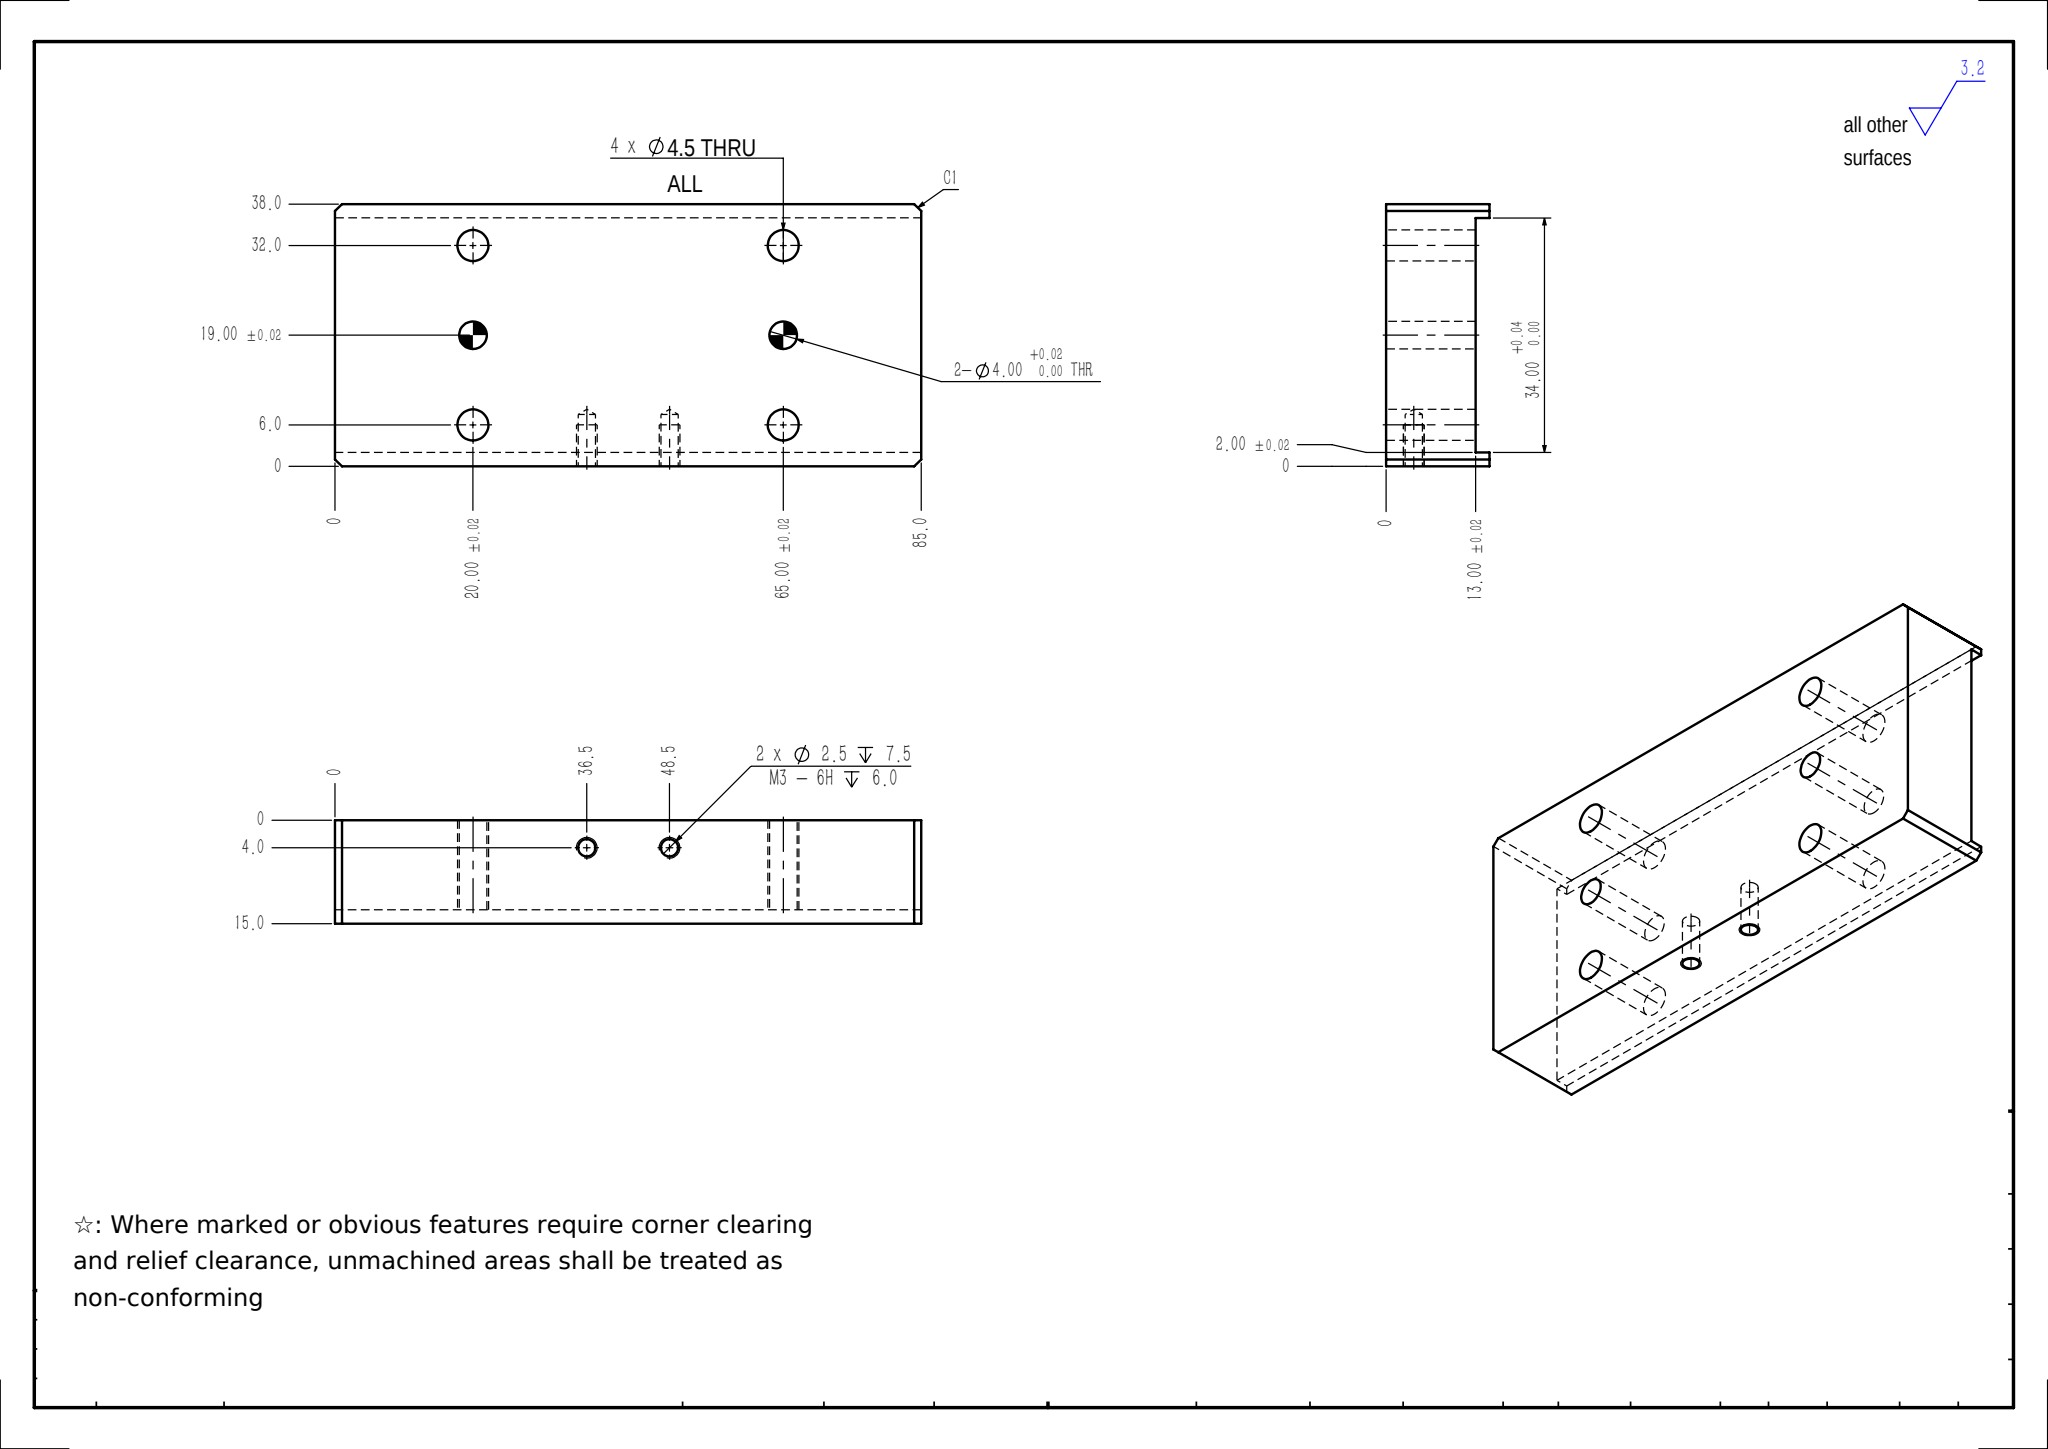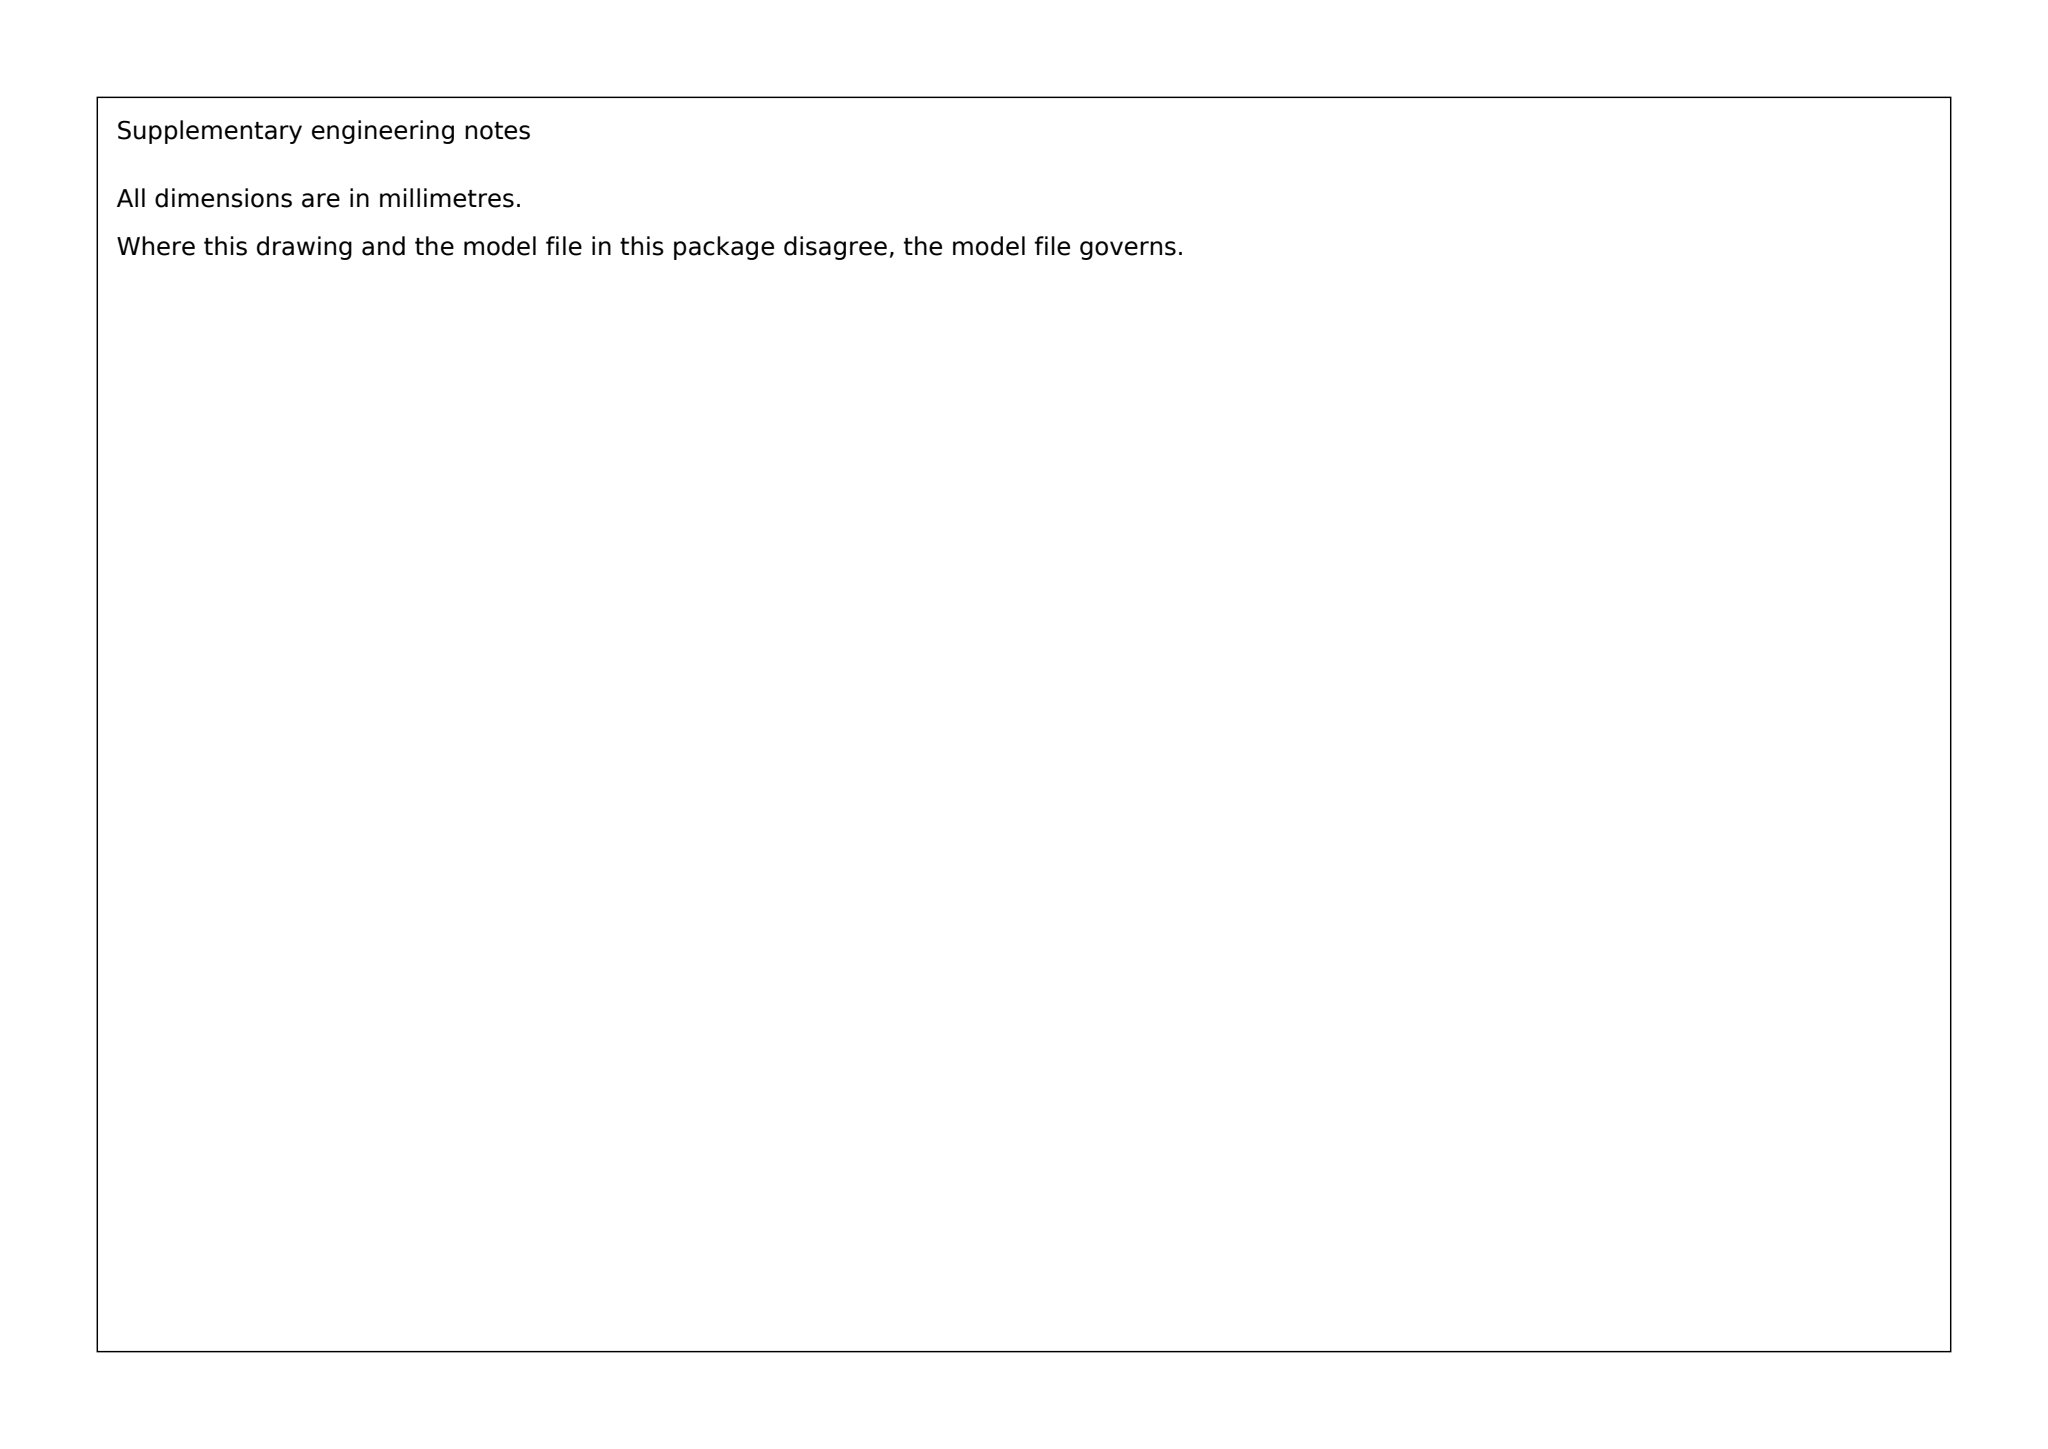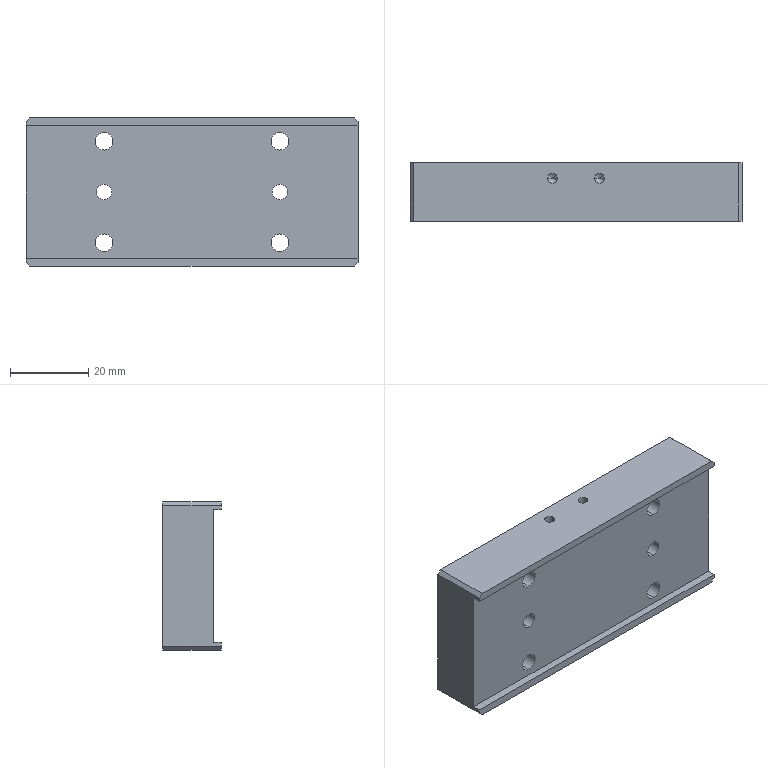Part | SolidWorks | mm | 1 solid | 34 faces | box 85 x 15 x 38 mm | volume 41410 mm3 | cylinder 16 | plane 14 | cone 4 | commonest cylinder face diameters 4.5 x8 2.5 x4 4 x4
Drawing notes:
2-Ø4.00 +0.02/0.00 THRU (13 THK WALL) | from the solid: Two Ø4.0 cylinders, axis Y at x=20.0 and 65.0, z=19.0, from y=2.0 to y=15.0 = full 13 wall thickness (face y=2 to face y=15)
2 x Ø4.00 +0.02/0.00 THRU, 19.00 UP, AT X=20.00 & 65.00 | from the solid: cylinders dia 4.0 axis y at (20,19) and (65,19), from y=2.0 to 15.0 (thru 13 wall)
build123d program:
from build123d import *

# Parameters (mm, degrees)
SKETCH1_W                 = 85
SKETCH1_H                 = 38
BOSS_EXTRUDE1_DEPTH       = 15
M4_CLEARANCE_HOLE1_D      = 4.5
SKETCH5_W                 = 85
SKETCH5_H                 = 34
CUT_EXTRUDE1_DEPTH        = 2
SIZE_MM_DOWEL_PIN_HOLE2_D = 4
CHAMFER1_SIZE             = 1
M3_TAPPED_HOLE1_D         = 2.5
M3_TAPPED_HOLE1_DEPTH     = 7.5
M3_TAPPED_HOLE1_TIP       = 0.7511


with BuildPart() as part:
    # Sketch1 → Boss-Extrude1 (new body)
    with BuildSketch(Plane(origin=(0, 0, 0), x_dir=(1, 0, 0), z_dir=(0, 1, 0))):
        Rectangle(SKETCH1_W, SKETCH1_H)
    extrude(amount=BOSS_EXTRUDE1_DEPTH)

    # M4 Clearance Hole1 (through all)
    with Locations(Plane(origin=(0, 15, 0), x_dir=(1, 0, 0), z_dir=(0, 1, 0))):
        with Locations((-22.5, 13), (-22.5, -13), (22.5, -13), (22.5, 13)):
            Hole(M4_CLEARANCE_HOLE1_D / 2)

    # Sketch5 → Cut-Extrude1 (cut)
    with BuildSketch(Plane.XZ):
        Rectangle(SKETCH5_W, SKETCH5_H)
    extrude(amount=-CUT_EXTRUDE1_DEPTH, mode=Mode.SUBTRACT)

    # Size mm Dowel Pin Hole2 (through all)
    with Locations(Plane(origin=(0, 15, 0), x_dir=(1, 0, 0), z_dir=(0, 1, 0))):
        with Locations((22.5, 0), (-22.5, 0)):
            Hole(SIZE_MM_DOWEL_PIN_HOLE2_D / 2)

    # Chamfer1
    chamfer1_edges = [part.edges().sort_by_distance(p)[0] for p in [
        (-42.5, 7.5, -19),
        (42.5, 7.5, -19),
        (42.5, 7.5, 19),
        (-42.5, 7.5, 19),
    ]]
    chamfer(chamfer1_edges, length=CHAMFER1_SIZE)

    # M3 Tapped Hole1
    with Locations(Plane.XY.offset(19)):
        with Locations((-6, 11), (6, 11)):
            Hole(M3_TAPPED_HOLE1_D / 2, depth=M3_TAPPED_HOLE1_DEPTH)
            with Locations((0, 0, -(M3_TAPPED_HOLE1_DEPTH + M3_TAPPED_HOLE1_TIP / 2))):  # 118° drill point
                Cone(0, M3_TAPPED_HOLE1_D / 2, M3_TAPPED_HOLE1_TIP, mode=Mode.SUBTRACT)


solid = part.part